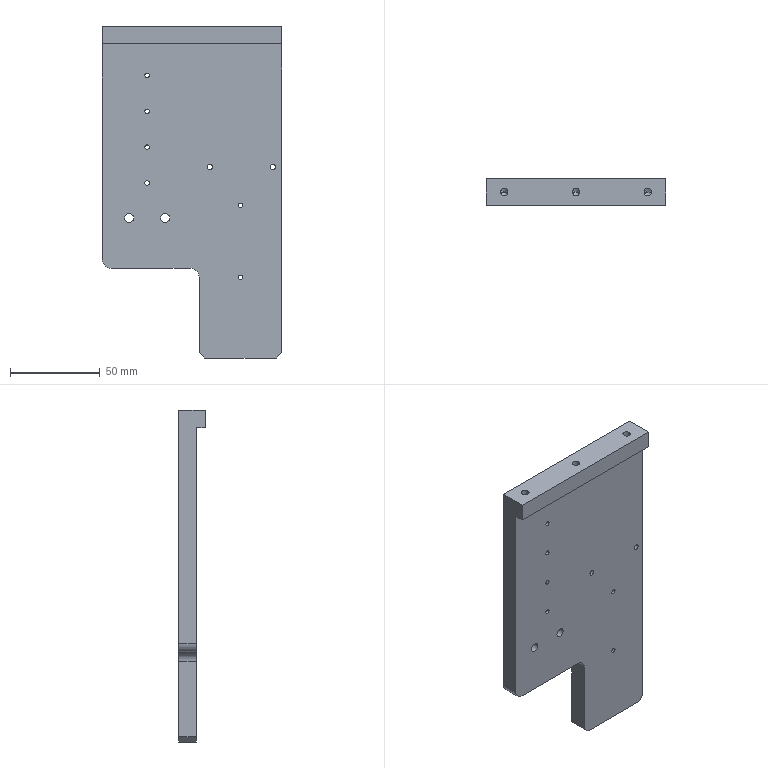Component | SolidWorks | P-SLJ-002-2_P-SLJ-002-001-1 | 1 solid | 54 faces | box 100 x 15 x 185 mm | volume 161082 mm3 | cylinder 32 | plane 12 | cone 10 | commonest cylinder face diameters 2.5 x12 4.2 x10 5 x4 3 x4 10 x2 | material Al 6061
build123d program:
from build123d import *

# Parameters (mm, degrees)
EXTRUDE1_DEPTH            = 50
M3_TAPPED_HOLE1_D         = 2.5
M3_TAPPED_HOLE2_D         = 2.5
SKETCH10_W                = 50
SKETCH10_H                = 54
CUT_EXTRUDE1_DEPTH        = 192.898
FILLET1_R                 = 5
SKETCH11_W                = 5
SKETCH11_H                = 5
EXTRUDE2_DEPTH            = 211.832
SKETCH12_W                = 10
SKETCH12_H                = 5
EXTRUDE3_DEPTH            = 100
M5_TAPPED_HOLE2_D         = 4.2
M5_TAPPED_HOLE2_DEPTH     = 14
M5_TAPPED_HOLE2_TIP       = 1.262
SIZE_MM_DOWEL_PIN_HOLE1_D = 3
M5_TAPPED_HOLE3_D         = 4.2
M5_TAPPED_HOLE3_DEPTH     = 14
M5_TAPPED_HOLE3_TIP       = 1.262
CHAMFER1_SIZE             = 3
M6_TAPPED_HOLE1_D         = 5


with BuildPart() as part:
    # Sketch1 → Extrude1 (new, symmetric)
    with BuildSketch(Plane.XY):
        Polygon((0, 0), (185, 0), (185, 10), (5, 10), (5, 15), (0, 15), align=None)
    extrude(amount=EXTRUDE1_DEPTH, both=True)

    # M3 Tapped Hole1 (through all)
    with Locations(Plane(origin=(0, 10, 0), x_dir=(1, 0, 0), z_dir=(0, 1, 0))):
        with Locations((100, -27), (140, -27)):
            Hole(M3_TAPPED_HOLE1_D / 2)

    # M3 Tapped Hole2 (through all)
    with Locations(Plane(origin=(0, 10, 0), x_dir=(1, 0, 0), z_dir=(0, 1, 0))):
        with Locations((27.5, 25), (47.5, 25), (67.5, 25), (87.5, 25)):
            Hole(M3_TAPPED_HOLE2_D / 2)

    # Sketch10 → Cut-Extrude1 (cut, through all)
    with BuildSketch(Plane(origin=(0, 10, 0), x_dir=(1, 0, 0), z_dir=(0, 1, 0))):
        with Locations((160, 23)):
            Rectangle(SKETCH10_W, SKETCH10_H)
    extrude(amount=-CUT_EXTRUDE1_DEPTH, mode=Mode.SUBTRACT)

    # Fillet1
    fillet1_edges = [part.edges().sort_by_distance(p)[0] for p in [
        (135, 5, 4),
        (135, 5, -50),
    ]]
    fillet(fillet1_edges, radius=FILLET1_R)

    # Sketch11 → Extrude2 (cut, through all)
    with BuildSketch(Plane.XY.offset(50)):
        with Locations((2.5, 12.5)):
            Rectangle(SKETCH11_W, SKETCH11_H)
    extrude(amount=-EXTRUDE2_DEPTH, mode=Mode.SUBTRACT)

    # Sketch12 → Extrude3 (add, through all)
    with BuildSketch(Plane.XY.offset(50)):
        with Locations((5, -2.5)):
            Rectangle(SKETCH12_W, SKETCH12_H)
    extrude(amount=-EXTRUDE3_DEPTH)

    # M5 Tapped Hole2
    with Locations(Plane.ZY):
        with Locations((40, 2.5), (0, 2.5), (-40, 2.5)):
            Hole(M5_TAPPED_HOLE2_D / 2, depth=M5_TAPPED_HOLE2_DEPTH)
            with Locations((0, 0, -(M5_TAPPED_HOLE2_DEPTH + M5_TAPPED_HOLE2_TIP / 2))):  # 118° drill point
                Cone(0, M5_TAPPED_HOLE2_D / 2, M5_TAPPED_HOLE2_TIP, mode=Mode.SUBTRACT)

    # Size mm Dowel Pin Hole1 (through all)
    with Locations(Plane(origin=(0, 10, 0), x_dir=(1, 0, 0), z_dir=(0, 1, 0))):
        with Locations((78.5, -45), (78.5, -10)):
            Hole(SIZE_MM_DOWEL_PIN_HOLE1_D / 2)

    # M5 Tapped Hole3
    with Locations(Plane(origin=(185, 0, 0), x_dir=(0, 0, -1), z_dir=(1, 0, 0))):
        with Locations((-42, 5), (-12, 5)):
            Hole(M5_TAPPED_HOLE3_D / 2, depth=M5_TAPPED_HOLE3_DEPTH)
            with Locations((0, 0, -(M5_TAPPED_HOLE3_DEPTH + M5_TAPPED_HOLE3_TIP / 2))):  # 118° drill point
                Cone(0, M5_TAPPED_HOLE3_D / 2, M5_TAPPED_HOLE3_TIP, mode=Mode.SUBTRACT)

    # Chamfer1
    chamfer1_edges = [part.edges().sort_by_distance(p)[0] for p in [
        (185, 5, 50),
        (185, 5, 4),
    ]]
    chamfer(chamfer1_edges, length=CHAMFER1_SIZE)

    # M6 Tapped Hole1 (through all)
    with Locations(Plane(origin=(0, 0, 0), x_dir=(-1, 0, 0), z_dir=(0, -1, 0))):
        with Locations((-107, 35), (-107, 15)):
            Hole(M6_TAPPED_HOLE1_D / 2)


solid = part.part

# Placed as in the assembly
solid = solid.moved(Location((-220, -83, 991.634), (0, 90, 0)))